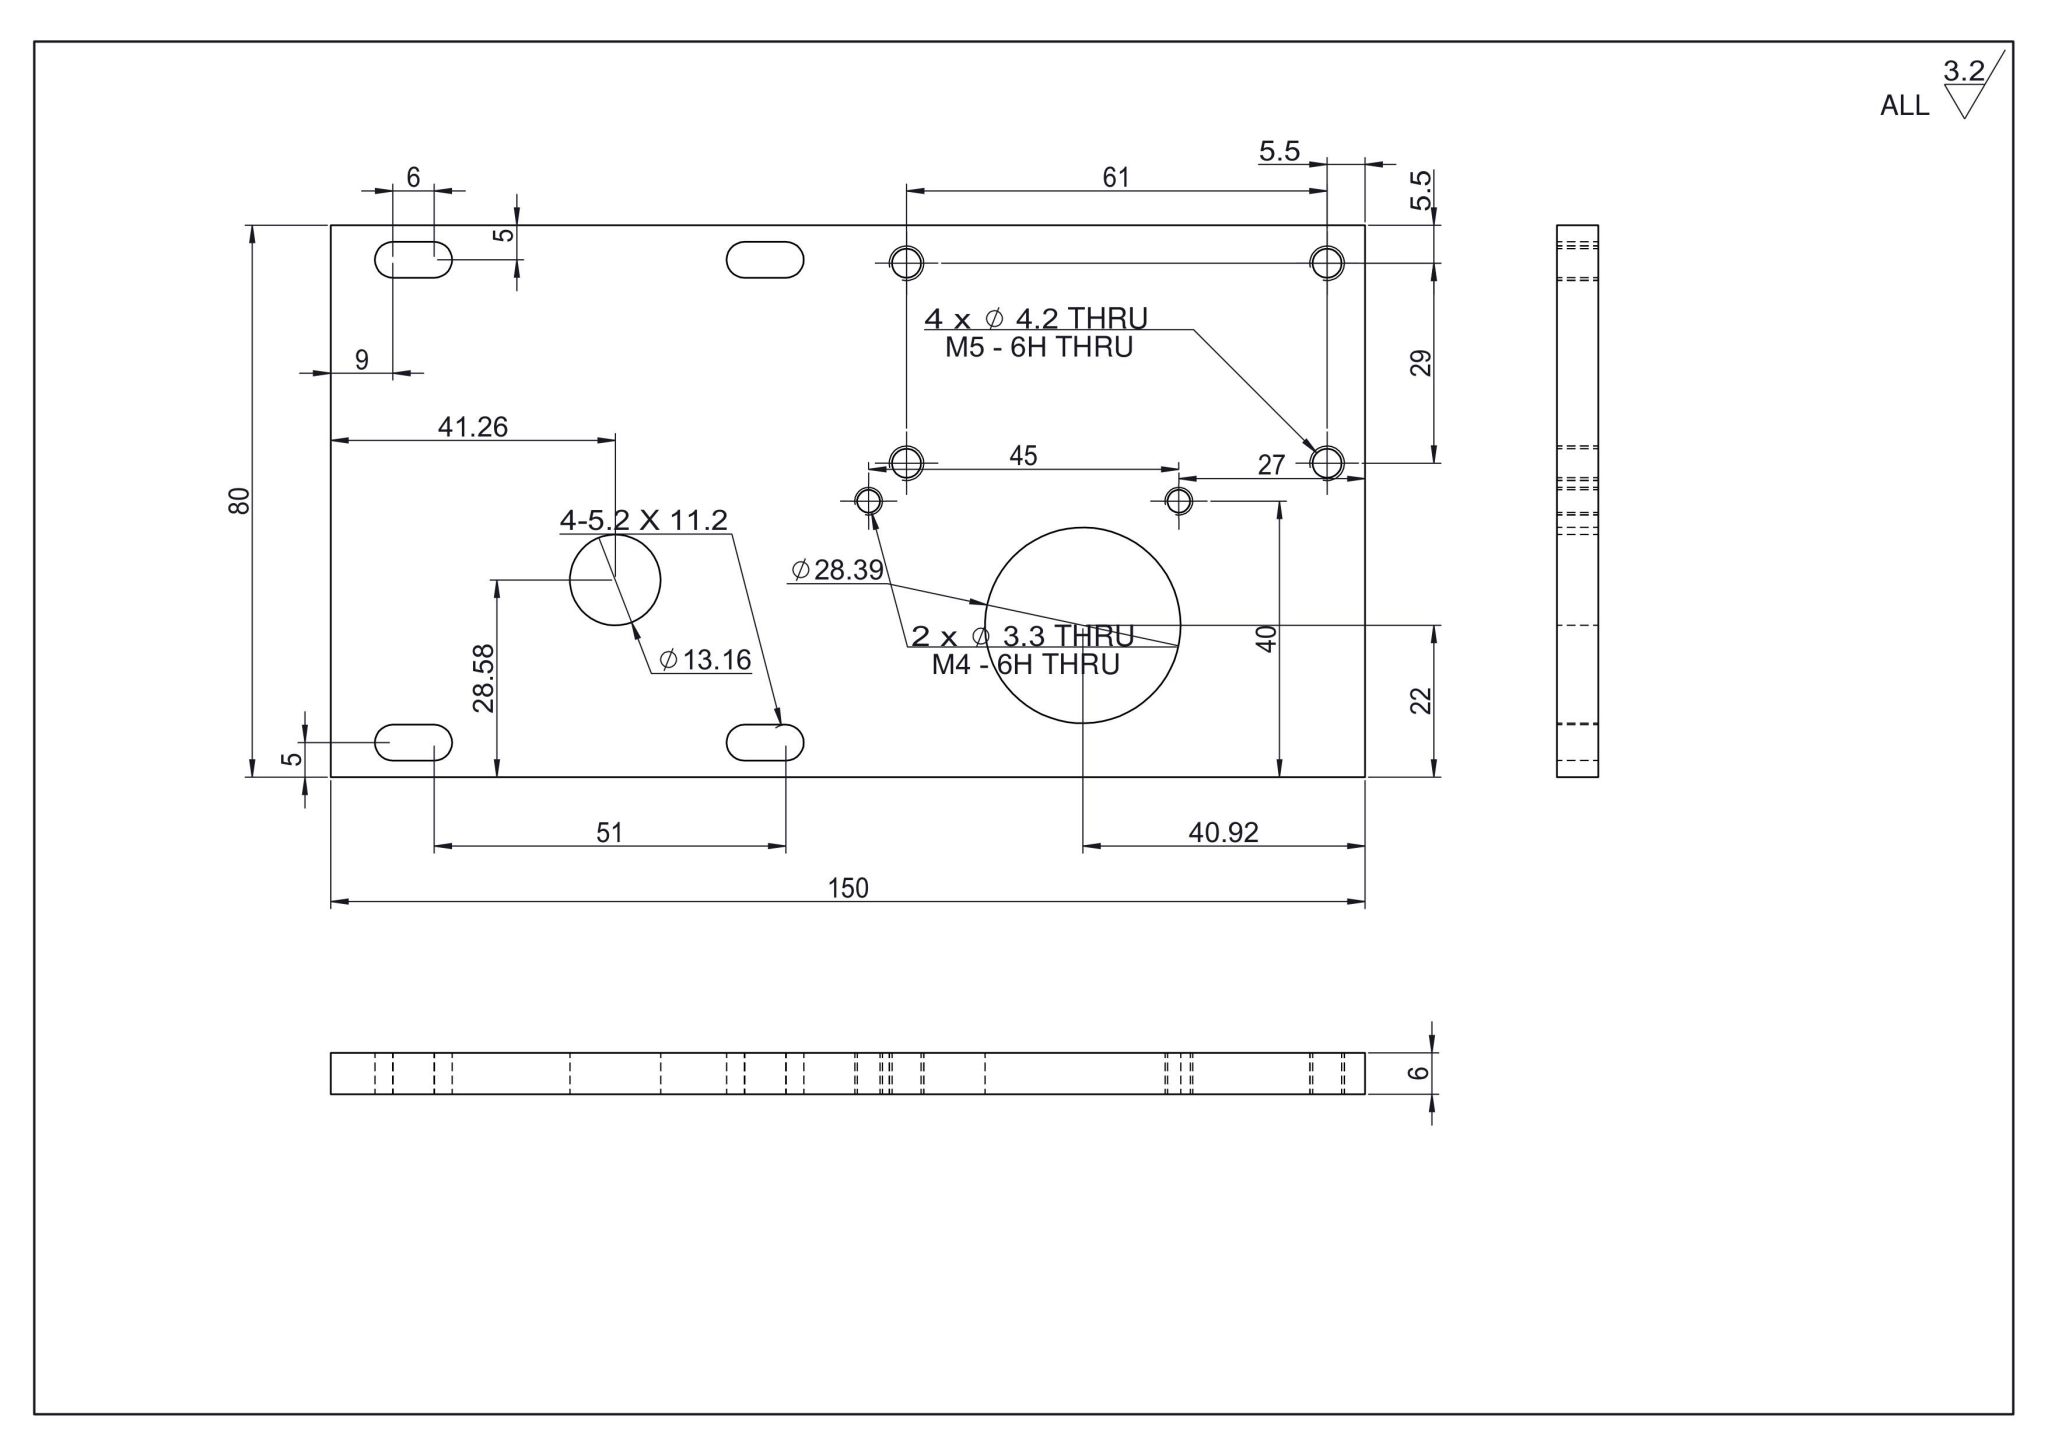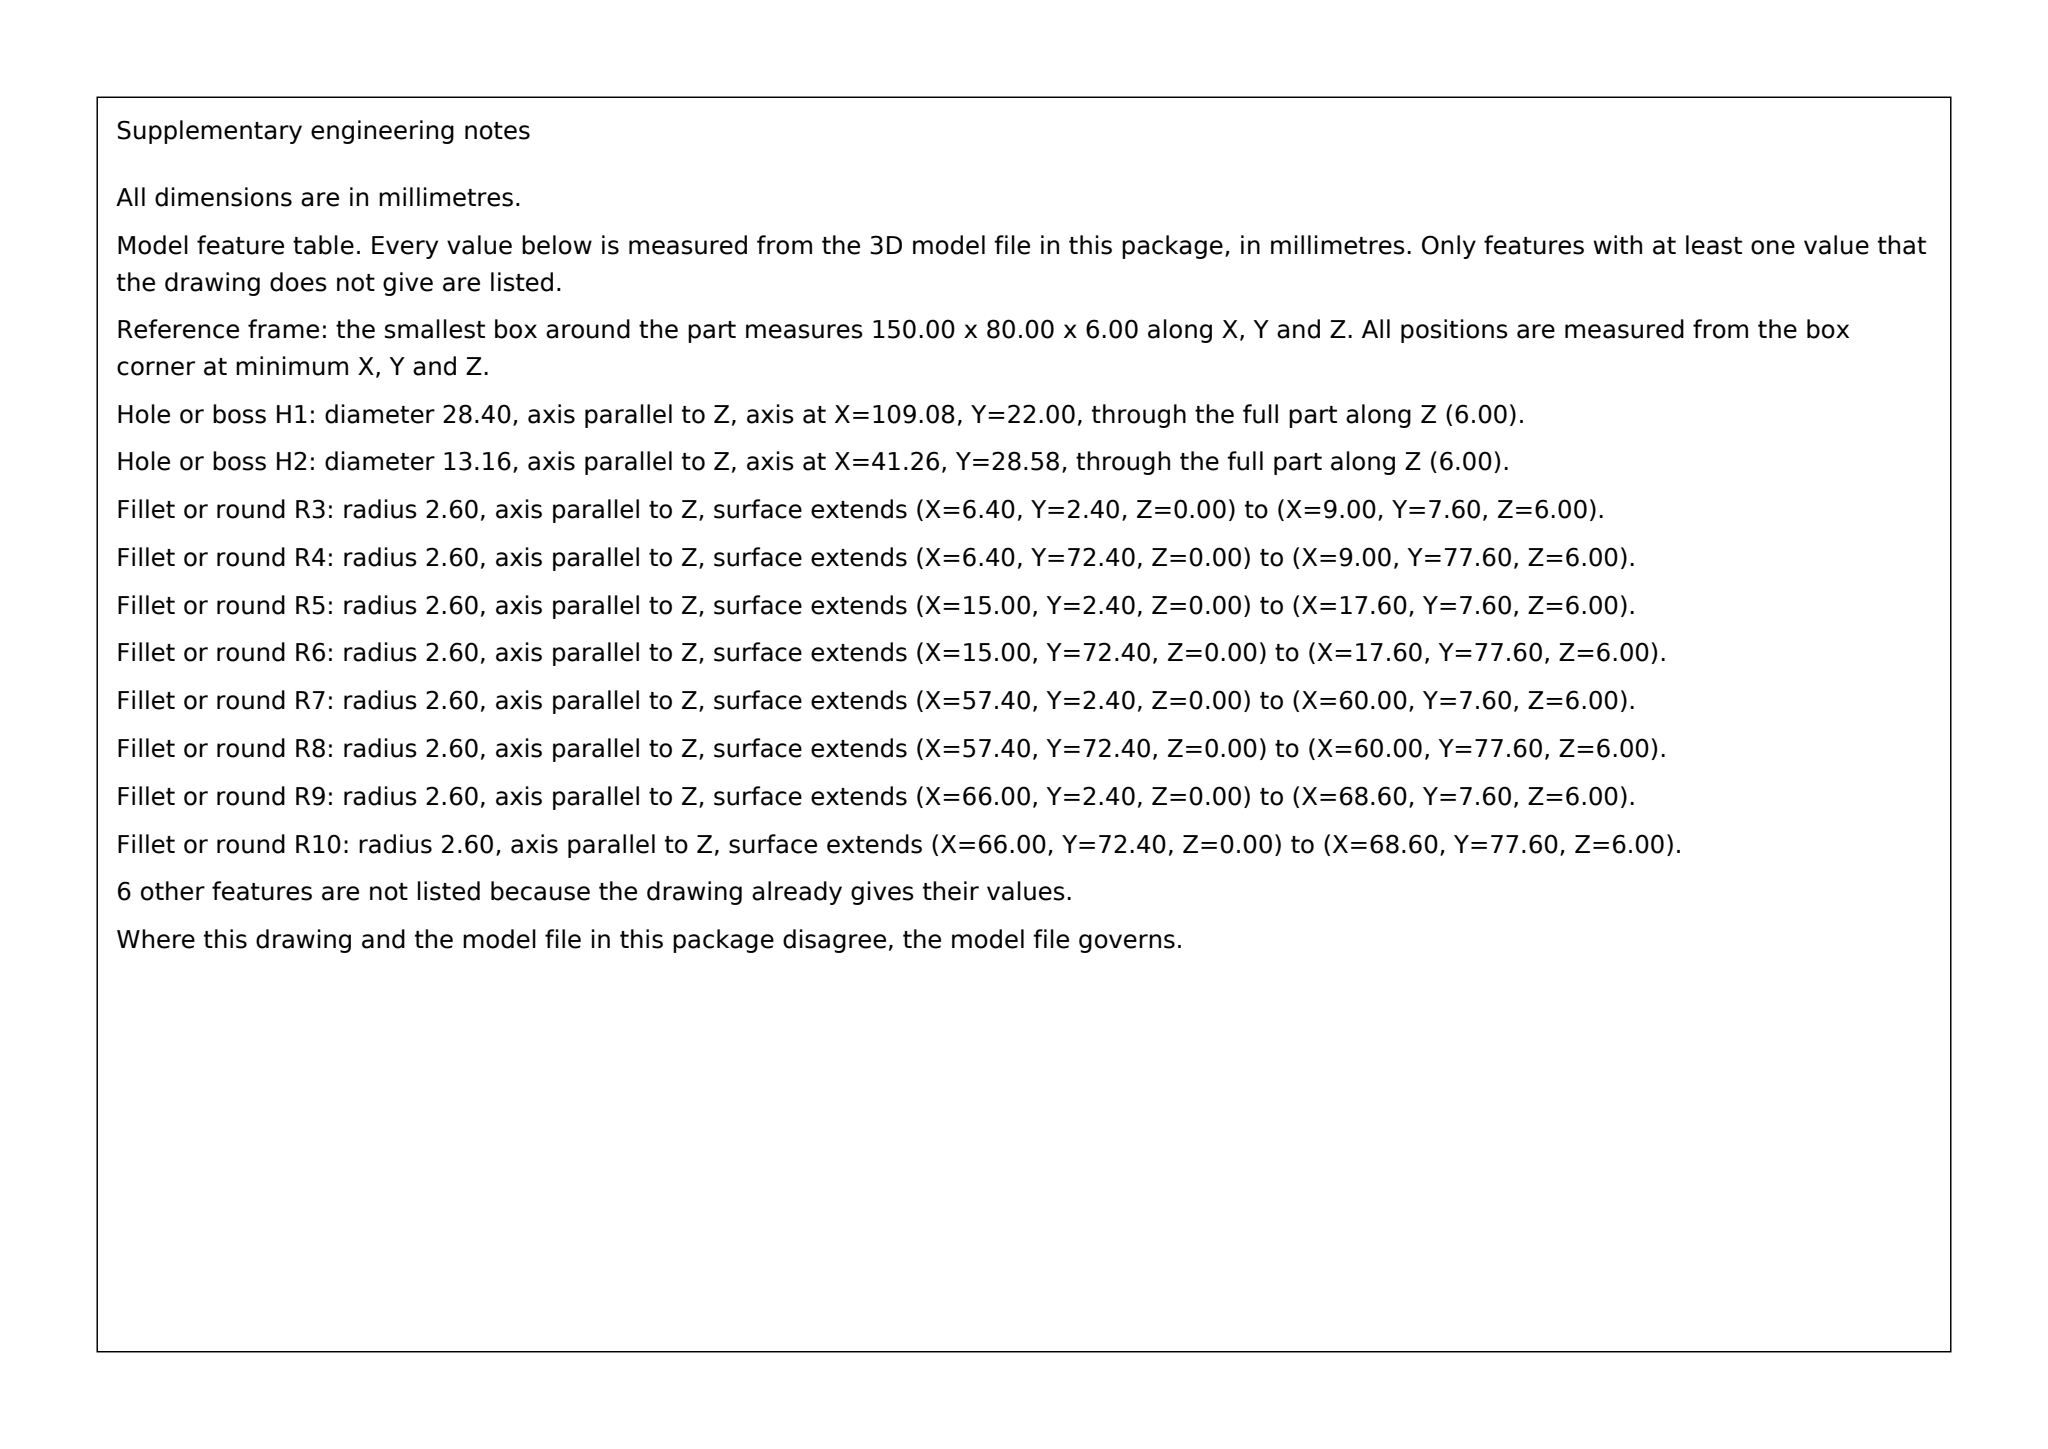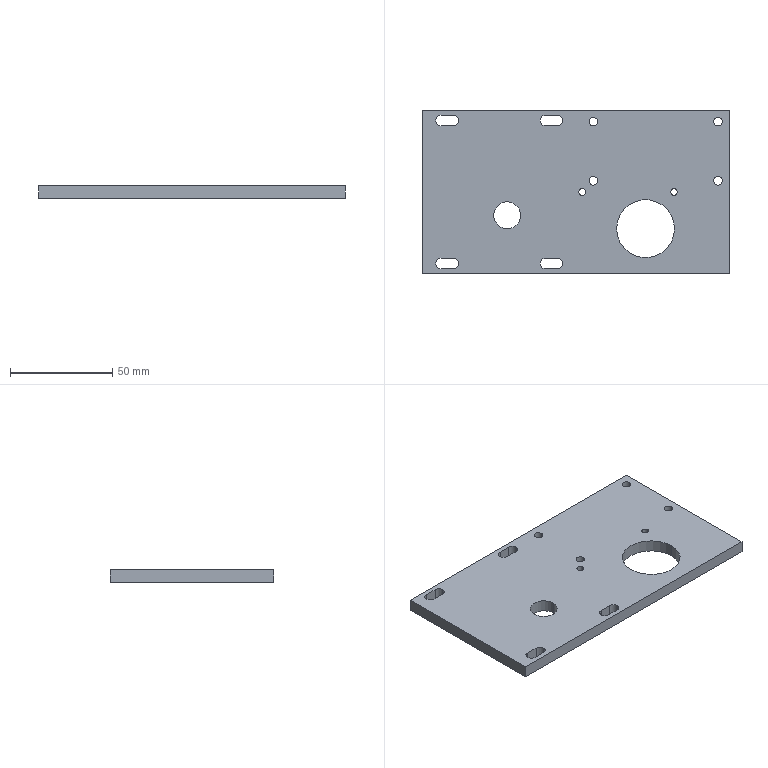Part | SolidWorks | mm | 1 solid | 42 faces | box 150 x 80 x 6 mm | volume 65691 mm3 | cylinder 28 | plane 14 | commonest cylinder face diameters 5.2 x12 4.2 x8 3.3 x4 13.162 x2 28.391 x2
build123d program:
from build123d import *

# Parameters (mm, degrees)
SKETCH1_W           = 150
SKETCH1_H           = 80
BOSS_EXTRUDE1_DEPTH = 6
CUT_EXTRUDE1_DEPTH  = 171.106
M4_TAPPED_HOLE1_D   = 3.3
M5_TAPPED_HOLE1_D   = 4.2
SKETCH7_R           = 6.581
SKETCH7_R_2         = 14.196
CUT_EXTRUDE2_DEPTH  = 80


with BuildPart() as part:
    # Sketch1 → Boss-Extrude1 (new body)
    with BuildSketch(Plane.XY):
        with Locations((75, 40)):
            Rectangle(SKETCH1_W, SKETCH1_H)
    extrude(amount=BOSS_EXTRUDE1_DEPTH)

    # Sketch2 → Cut-Extrude1 (cut, through all)
    with BuildSketch(Plane.XY.offset(6)):
        with BuildLine():
            Line((9, 77.6), (15, 77.6))
            ThreePointArc((15, 77.6), (17.6, 75), (15, 72.4))
            Line((15, 72.4), (9, 72.4))
            ThreePointArc((9, 72.4), (6.4, 75), (9, 77.6))
        make_face()
        with BuildLine():
            Line((60, 77.6), (66, 77.6))
            ThreePointArc((66, 77.6), (68.6, 75), (66, 72.4))
            Line((66, 72.4), (60, 72.4))
            ThreePointArc((60, 72.4), (57.4, 75), (60, 77.6))
        make_face()
        with BuildLine():
            Line((9, 7.6), (15, 7.6))
            ThreePointArc((15, 7.6), (17.6, 5), (15, 2.4))
            Line((15, 2.4), (9, 2.4))
            ThreePointArc((9, 2.4), (6.4, 5), (9, 7.6))
        make_face()
        with BuildLine():
            Line((60, 7.6), (66, 7.6))
            ThreePointArc((66, 7.6), (68.6, 5), (66, 2.4))
            Line((66, 2.4), (60, 2.4))
            ThreePointArc((60, 2.4), (57.4, 5), (60, 7.6))
        make_face()
    extrude(amount=-CUT_EXTRUDE1_DEPTH, mode=Mode.SUBTRACT)

    # M4 Tapped Hole1 (through all)
    with Locations(Plane.XY.offset(6)):
        with Locations((78, 40), (123, 40)):
            Hole(M4_TAPPED_HOLE1_D / 2)

    # M5 Tapped Hole1 (through all)
    with Locations(Plane(origin=(0, 0, 0), x_dir=(-1, 0, 0), z_dir=(0, 0, -1))):
        with Locations((-144.5, 45.5), (-144.5, 74.5), (-83.5, 74.5), (-83.5, 45.5)):
            Hole(M5_TAPPED_HOLE1_D / 2)

    # Sketch7 → Cut-Extrude2 (cut)
    with BuildSketch(Plane.XY.offset(6)):
        with Locations((41.265, 28.585)):
            Circle(SKETCH7_R)
        with Locations((109.076, 22.003)):
            Circle(SKETCH7_R_2)
    extrude(amount=-CUT_EXTRUDE2_DEPTH, mode=Mode.SUBTRACT)


solid = part.part